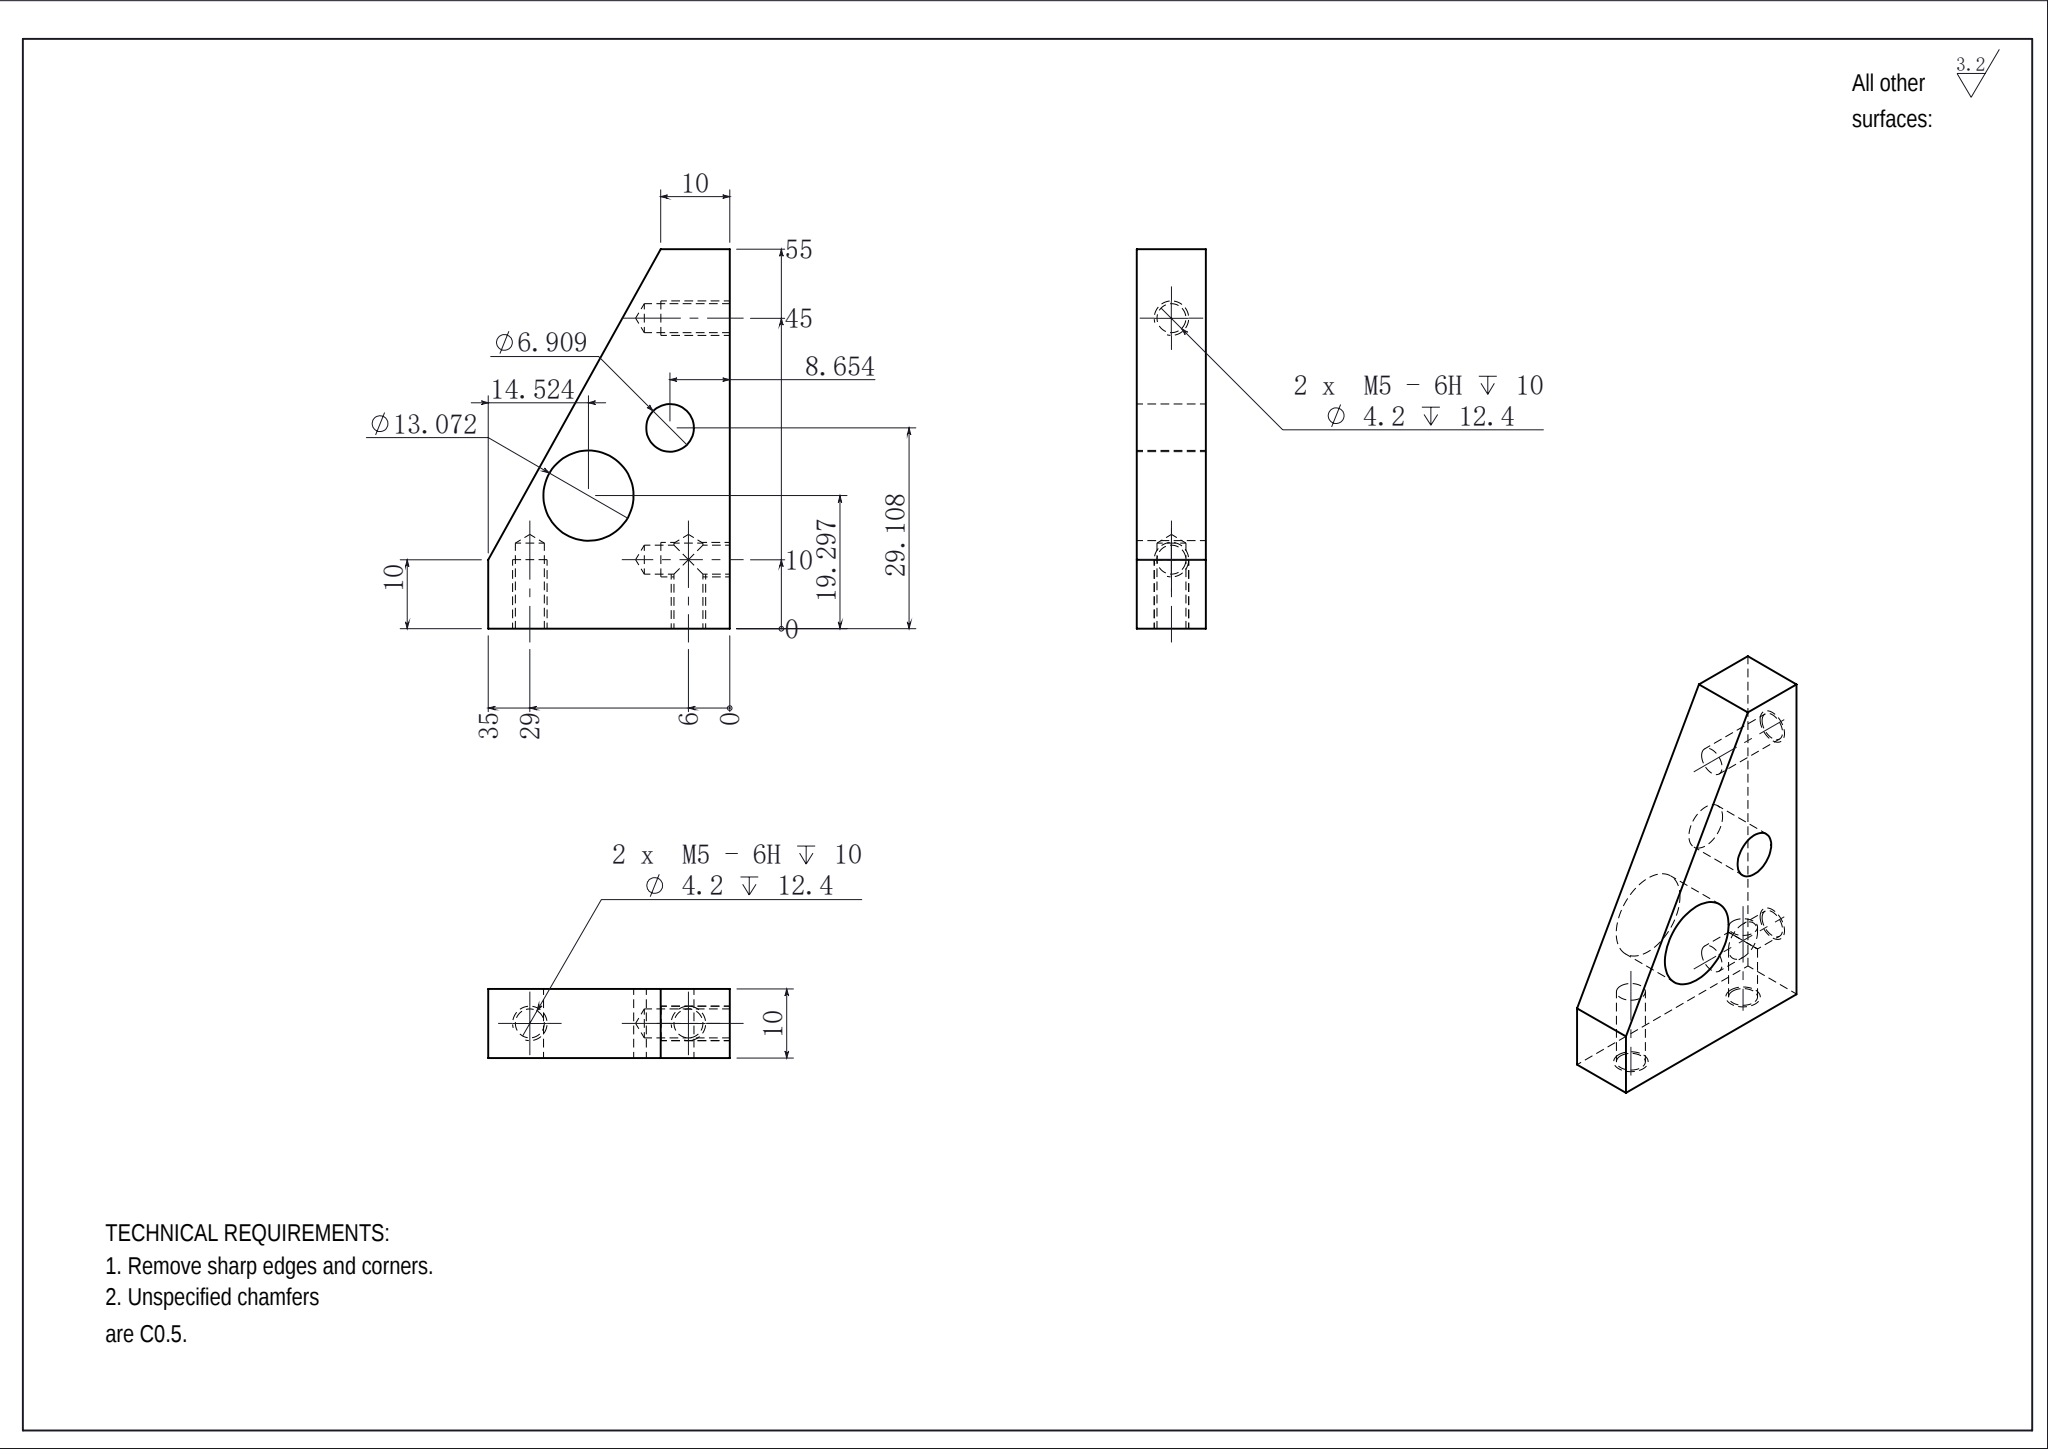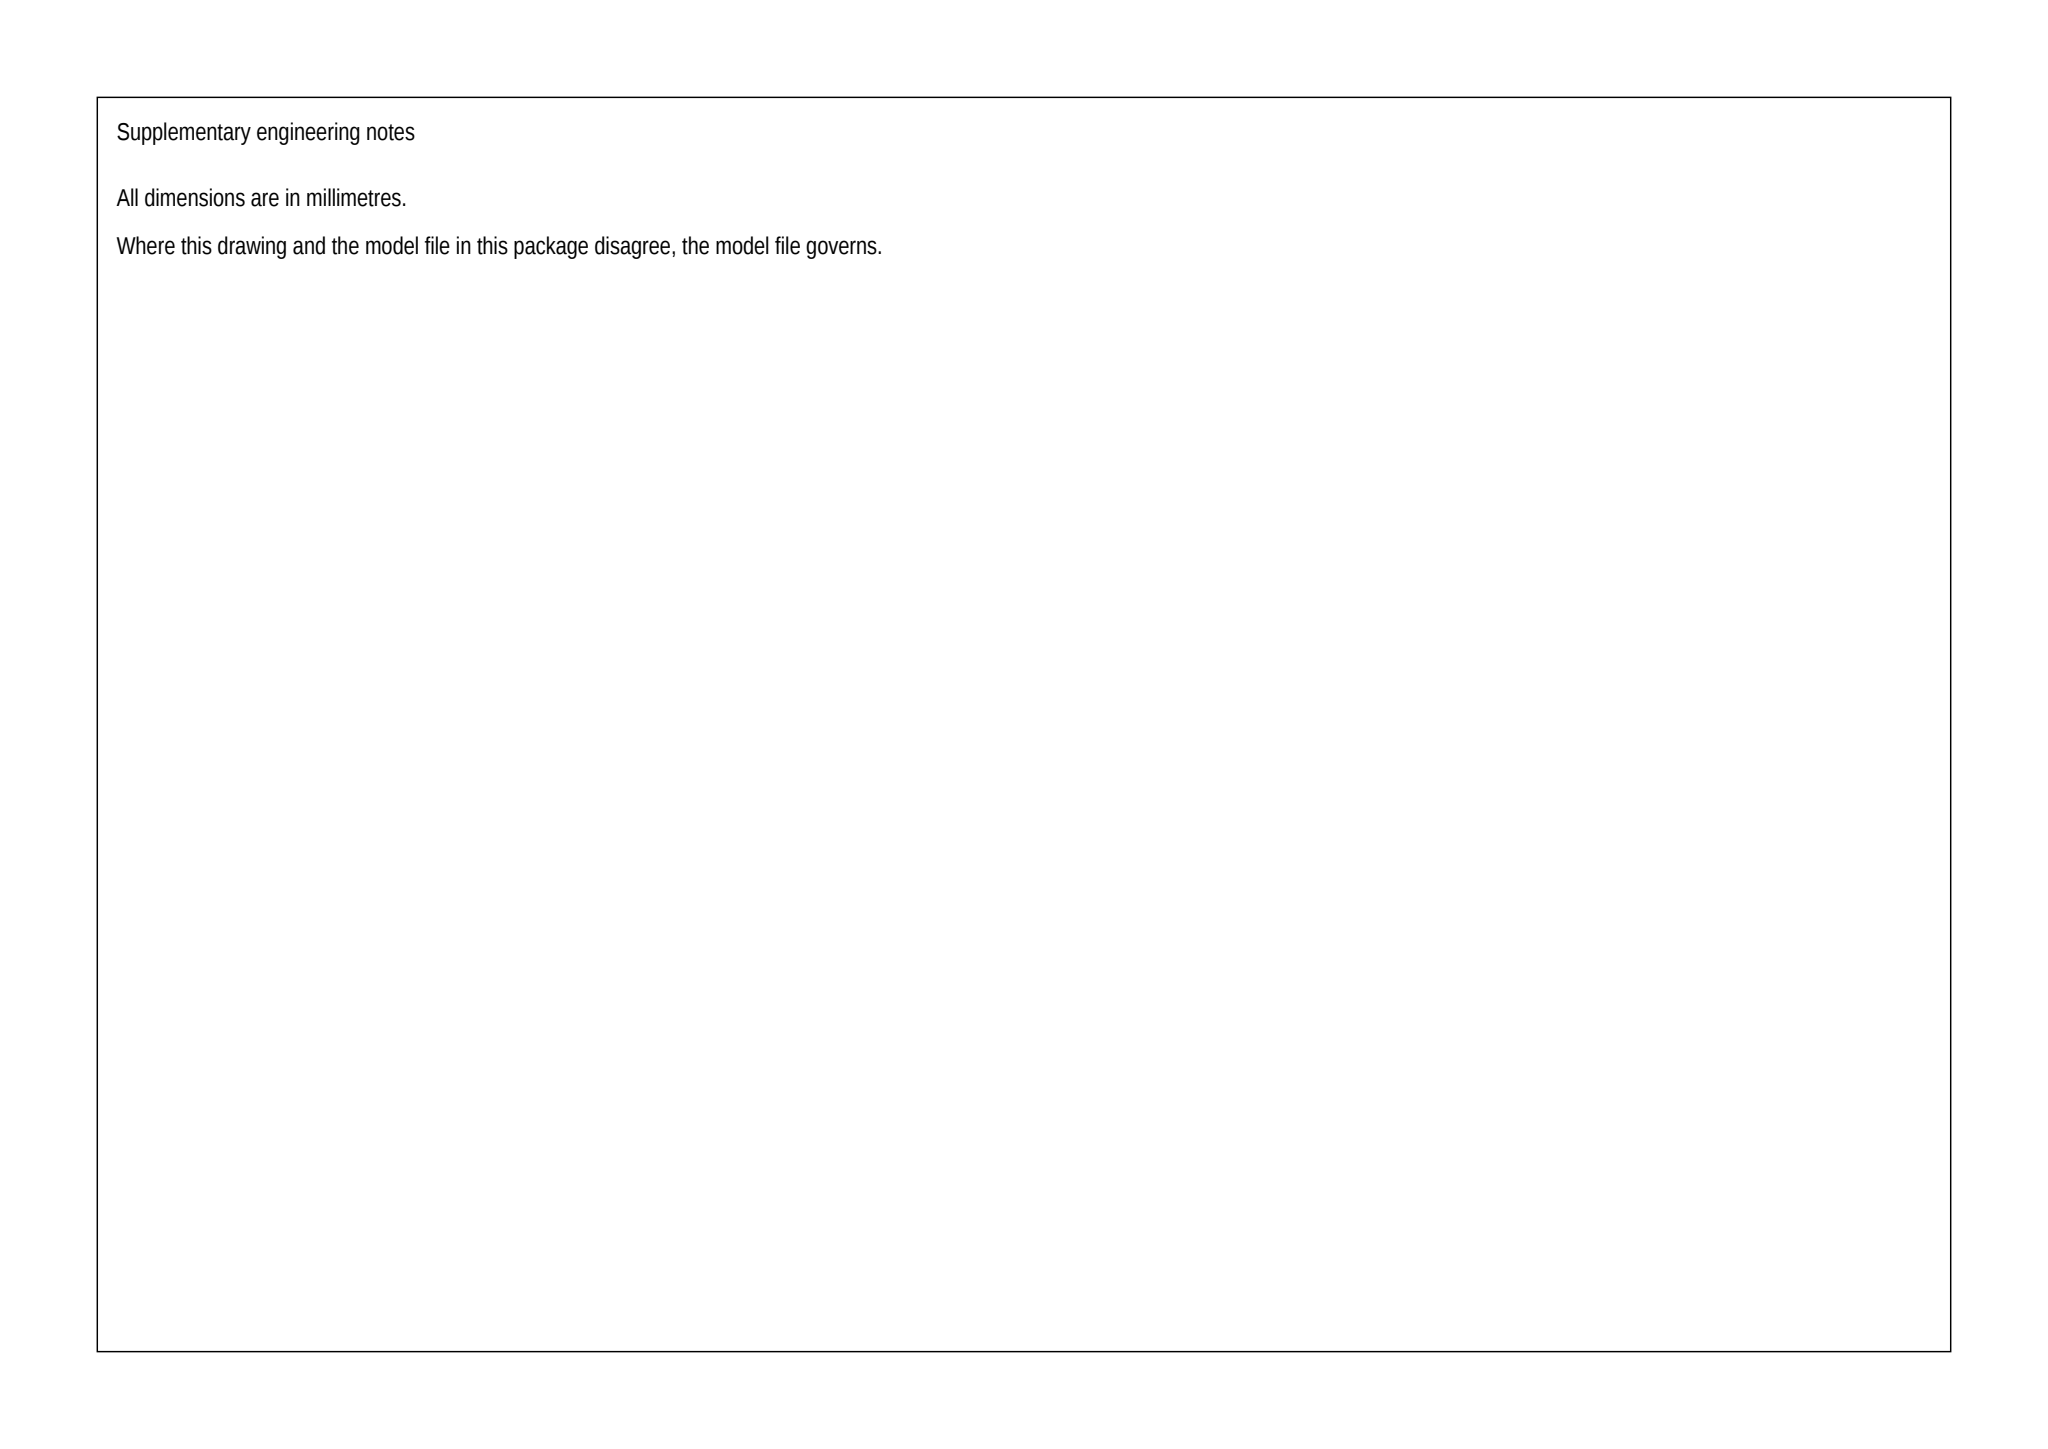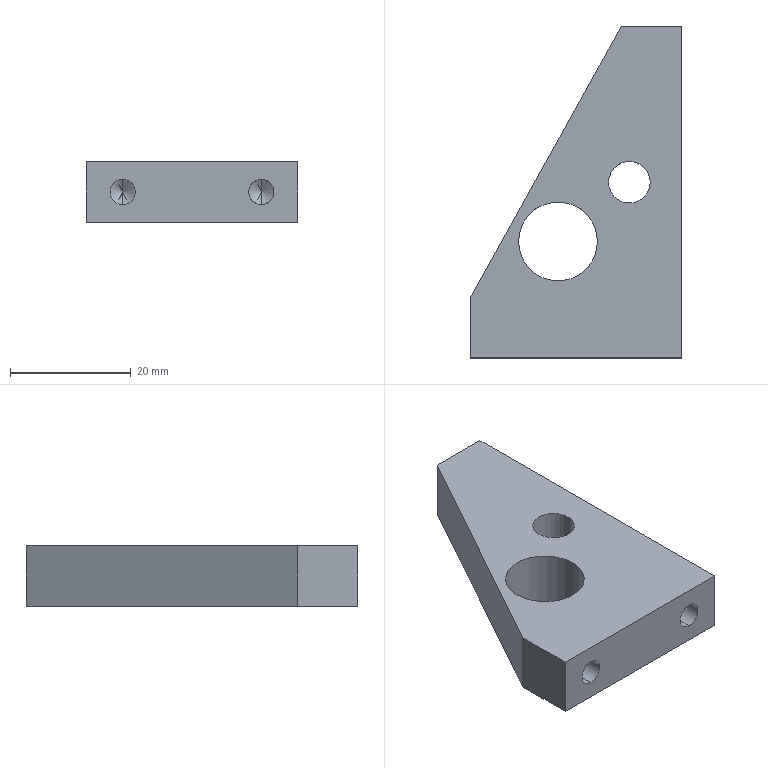Part | SolidWorks | mm | 1 solid | 31 faces | box 35 x 55 x 10 mm | volume 11247 mm3 | cylinder 16 | cone 8 | plane 7 | commonest cylinder face diameters 4.2 x12 13.072 x2 6.909 x2
build123d program:
from build123d import *

# Parameters (mm, degrees)
BOSS_EXTRUDE1_DEPTH   = 5
M5_TAPPED_HOLE1_D     = 4.2
M5_TAPPED_HOLE1_DEPTH = 12.4
M5_TAPPED_HOLE1_TIP   = 1.262
M5_TAPPED_HOLE2_D     = 4.2
M5_TAPPED_HOLE2_DEPTH = 12.4
M5_TAPPED_HOLE2_TIP   = 1.262
SKETCH7_R             = 6.536
SKETCH7_R_2           = 3.454
CUT_EXTRUDE1_DEPTH    = 80


with BuildPart() as part:
    # Sketch1 → Boss-Extrude1 (new, symmetric)
    with BuildSketch(Plane.XY):
        Polygon((0, 0), (0, 55), (-10, 55), (-35, 10), (-35, 0), align=None)
    extrude(amount=BOSS_EXTRUDE1_DEPTH, both=True)

    # M5 Tapped Hole1
    with Locations(Plane(origin=(0, 0, 0), x_dir=(0, 0, -1), z_dir=(1, 0, 0))):
        with Locations((0, 45), (0, 10)):
            Hole(M5_TAPPED_HOLE1_D / 2, depth=M5_TAPPED_HOLE1_DEPTH)
            with Locations((0, 0, -(M5_TAPPED_HOLE1_DEPTH + M5_TAPPED_HOLE1_TIP / 2))):  # 118° drill point
                Cone(0, M5_TAPPED_HOLE1_D / 2, M5_TAPPED_HOLE1_TIP, mode=Mode.SUBTRACT)

    # M5 Tapped Hole2
    with Locations(Plane(origin=(0, 0, 0), x_dir=(-1, 0, 0), z_dir=(0, -1, 0))):
        with Locations((6, 0), (29, 0)):
            Hole(M5_TAPPED_HOLE2_D / 2, depth=M5_TAPPED_HOLE2_DEPTH)
            with Locations((0, 0, -(M5_TAPPED_HOLE2_DEPTH + M5_TAPPED_HOLE2_TIP / 2))):  # 118° drill point
                Cone(0, M5_TAPPED_HOLE2_D / 2, M5_TAPPED_HOLE2_TIP, mode=Mode.SUBTRACT)

    # Sketch7 → Cut-Extrude1 (cut)
    with BuildSketch(Plane.XY.offset(5)):
        with Locations((-20.476, 19.297)):
            Circle(SKETCH7_R)
        with Locations((-8.654, 29.108)):
            Circle(SKETCH7_R_2)
    extrude(amount=-CUT_EXTRUDE1_DEPTH, mode=Mode.SUBTRACT)


solid = part.part
STEP:
#1=CARTESIAN_POINT('',(-27.011,19.297,-5.));
#2=VERTEX_POINT('',#1);
#3=CARTESIAN_POINT('',(-13.94,19.297,-5.));
#4=VERTEX_POINT('',#3);
#5=CARTESIAN_POINT('',(-20.476,19.297,-5.));
#6=DIRECTION('',(0.,0.,1.));
#7=DIRECTION('',(1.,0.,0.));
#8=AXIS2_PLACEMENT_3D('',#5,#6,#7);
#9=CIRCLE('',#8,6.536);
#10=EDGE_CURVE('',#2,#4,#9,.T.);
#11=ORIENTED_EDGE('',*,*,#10,.F.);
#12=CARTESIAN_POINT('',(-27.011,19.297,5.));
#13=VERTEX_POINT('',#12);
#14=CARTESIAN_POINT('',(-27.011,19.297,-75.));
#15=DIRECTION('',(0.,0.,1.));
#16=VECTOR('',#15,1000.);
#17=LINE('',#14,#16);
#18=EDGE_CURVE('',#2,#13,#17,.T.);
#19=ORIENTED_EDGE('',*,*,#18,.T.);
#20=CARTESIAN_POINT('',(-13.94,19.297,5.));
#21=VERTEX_POINT('',#20);
#22=CARTESIAN_POINT('',(-20.476,19.297,5.));
#23=DIRECTION('',(0.,0.,1.));
#24=DIRECTION('',(1.,0.,0.));
#25=AXIS2_PLACEMENT_3D('',#22,#23,#24);
#26=CIRCLE('',#25,6.536);
#27=EDGE_CURVE('',#13,#21,#26,.T.);
#28=ORIENTED_EDGE('',*,*,#27,.T.);
#29=CARTESIAN_POINT('',(-13.94,19.297,-75.));
#30=DIRECTION('',(0.,0.,1.));
#31=VECTOR('',#30,1000.);
#32=LINE('',#29,#31);
#33=EDGE_CURVE('',#4,#21,#32,.T.);
#34=ORIENTED_EDGE('',*,*,#33,.F.);
#35=EDGE_LOOP('',(#11,#19,#28,#34));
#36=FACE_OUTER_BOUND('',#35,.T.);
#37=CARTESIAN_POINT('',(-20.476,19.297,-75.));
#38=DIRECTION('',(0.,0.,1.));
#39=DIRECTION('',(1.,0.,0.));
#40=AXIS2_PLACEMENT_3D('',#37,#38,#39);
#41=CYLINDRICAL_SURFACE('',#40,6.536);
#42=ADVANCED_FACE('',(#36),#41,.F.);
#43=CARTESIAN_POINT('',(-12.108,29.108,-5.));
#44=VERTEX_POINT('',#43);
#45=CARTESIAN_POINT('',(-5.199,29.108,-5.));
#46=VERTEX_POINT('',#45);
#47=CARTESIAN_POINT('',(-8.654,29.108,-5.));
#48=DIRECTION('',(0.,0.,1.));
#49=DIRECTION('',(1.,0.,0.));
#50=AXIS2_PLACEMENT_3D('',#47,#48,#49);
#51=CIRCLE('',#50,3.454);
#52=EDGE_CURVE('',#44,#46,#51,.T.);
#53=ORIENTED_EDGE('',*,*,#52,.F.);
#54=CARTESIAN_POINT('',(-12.108,29.108,5.));
#55=VERTEX_POINT('',#54);
#56=CARTESIAN_POINT('',(-12.108,29.108,-75.));
#57=DIRECTION('',(0.,0.,1.));
#58=VECTOR('',#57,1000.);
#59=LINE('',#56,#58);
#60=EDGE_CURVE('',#44,#55,#59,.T.);
#61=ORIENTED_EDGE('',*,*,#60,.T.);
#62=CARTESIAN_POINT('',(-5.199,29.108,5.));
#63=VERTEX_POINT('',#62);
#64=CARTESIAN_POINT('',(-8.654,29.108,5.));
#65=DIRECTION('',(0.,0.,1.));
#66=DIRECTION('',(1.,0.,0.));
#67=AXIS2_PLACEMENT_3D('',#64,#65,#66);
#68=CIRCLE('',#67,3.454);
#69=EDGE_CURVE('',#55,#63,#68,.T.);
#70=ORIENTED_EDGE('',*,*,#69,.T.);
#71=CARTESIAN_POINT('',(-5.199,29.108,-75.));
#72=DIRECTION('',(0.,0.,1.));
#73=VECTOR('',#72,1000.);
#74=LINE('',#71,#73);
#75=EDGE_CURVE('',#46,#63,#74,.T.);
#76=ORIENTED_EDGE('',*,*,#75,.F.);
#77=EDGE_LOOP('',(#53,#61,#70,#76));
#78=FACE_OUTER_BOUND('',#77,.T.);
#79=CARTESIAN_POINT('',(-8.654,29.108,-75.));
#80=DIRECTION('',(0.,0.,1.));
#81=DIRECTION('',(1.,0.,0.));
#82=AXIS2_PLACEMENT_3D('',#79,#80,#81);
#83=CYLINDRICAL_SURFACE('',#82,3.454);
#84=ADVANCED_FACE('',(#78),#83,.F.);
#85=CARTESIAN_POINT('',(-6.,13.662,0.));
#86=VERTEX_POINT('',#85);
#87=CARTESIAN_POINT('',(-6.,12.4,-2.1));
#88=VERTEX_POINT('',#87);
#89=CARTESIAN_POINT('',(-6.,12.4,-2.1));
#90=DIRECTION('',(0.,-0.515,-0.8572));
#91=VECTOR('',#90,1000.);
#92=LINE('',#89,#91);
#93=EDGE_CURVE('',#86,#88,#92,.T.);
#94=ORIENTED_EDGE('',*,*,#93,.F.);
#95=CARTESIAN_POINT('',(-6.,12.4,2.1));
#96=VERTEX_POINT('',#95);
#97=CARTESIAN_POINT('',(-6.,12.4,2.1));
#98=DIRECTION('',(0.,-0.515,0.8572));
#99=VECTOR('',#98,1000.);
#100=LINE('',#97,#99);
#101=EDGE_CURVE('',#86,#96,#100,.T.);
#102=ORIENTED_EDGE('',*,*,#101,.T.);
#103=CARTESIAN_POINT('',(-6.,12.4,0.));
#104=DIRECTION('',(0.,-1.,0.));
#105=DIRECTION('',(0.,0.,-1.));
#106=AXIS2_PLACEMENT_3D('',#103,#104,#105);
#107=CIRCLE('',#106,2.1);
#108=EDGE_CURVE('',#96,#88,#107,.T.);
#109=ORIENTED_EDGE('',*,*,#108,.T.);
#110=EDGE_LOOP('',(#94,#102,#109));
#111=FACE_OUTER_BOUND('',#110,.T.);
#112=CARTESIAN_POINT('',(-6.,12.4,0.));
#113=DIRECTION('',(0.,-1.,0.));
#114=DIRECTION('',(0.,0.,-1.));
#115=AXIS2_PLACEMENT_3D('',#112,#113,#114);
#116=CONICAL_SURFACE('',#115,2.1,1.03);
#117=ADVANCED_FACE('',(#111),#116,.F.);
#118=ORIENTED_EDGE('',*,*,#108,.F.);
#119=CARTESIAN_POINT('',(-6.,10.,2.1));
#120=VERTEX_POINT('',#119);
#121=CARTESIAN_POINT('',(-6.,0.,2.1));
#122=DIRECTION('',(0.,-1.,0.));
#123=VECTOR('',#122,1000.);
#124=LINE('',#121,#123);
#125=EDGE_CURVE('',#96,#120,#124,.T.);
#126=ORIENTED_EDGE('',*,*,#125,.T.);
#127=CARTESIAN_POINT('',(-6.,10.,-2.1));
#128=VERTEX_POINT('',#127);
#129=CARTESIAN_POINT('',(-6.,10.,-2.1));
#130=CARTESIAN_POINT('',(-10.2,14.2,-2.1));
#131=CARTESIAN_POINT('',(-10.2,14.2,2.1));
#132=CARTESIAN_POINT('',(-6.,10.,2.1));
#133=(BOUNDED_CURVE()B_SPLINE_CURVE(3,(#129,#130,#131,#132),.UNSPECIFIED.,.F.,.F.)B_SPLINE_CURVE_WITH_KNOTS((4,4),(1.571,4.712),.UNSPECIFIED.)CURVE()GEOMETRIC_REPRESENTATION_ITEM()RATIONAL_B_SPLINE_CURVE((1.,0.3333,0.3333,1.))REPRESENTATION_ITEM(''));
#134=EDGE_CURVE('',#128,#120,#133,.T.);
#135=ORIENTED_EDGE('',*,*,#134,.F.);
#136=CARTESIAN_POINT('',(-6.,0.,-2.1));
#137=DIRECTION('',(0.,-1.,0.));
#138=VECTOR('',#137,1000.);
#139=LINE('',#136,#138);
#140=EDGE_CURVE('',#88,#128,#139,.T.);
#141=ORIENTED_EDGE('',*,*,#140,.F.);
#142=EDGE_LOOP('',(#118,#126,#135,#141));
#143=FACE_OUTER_BOUND('',#142,.T.);
#144=CARTESIAN_POINT('',(-6.,0.,0.));
#145=DIRECTION('',(0.,-1.,0.));
#146=DIRECTION('',(0.,0.,-1.));
#147=AXIS2_PLACEMENT_3D('',#144,#145,#146);
#148=CYLINDRICAL_SURFACE('',#147,2.1);
#149=ADVANCED_FACE('',(#143),#148,.F.);
#150=CARTESIAN_POINT('',(-12.4,10.,2.1));
#151=VERTEX_POINT('',#150);
#152=CARTESIAN_POINT('',(-12.4,10.,-2.1));
#153=VERTEX_POINT('',#152);
#154=CARTESIAN_POINT('',(-12.4,10.,-0.));
#155=DIRECTION('',(1.,0.,0.));
#156=DIRECTION('',(0.,0.,-1.));
#157=AXIS2_PLACEMENT_3D('',#154,#155,#156);
#158=CIRCLE('',#157,2.1);
#159=EDGE_CURVE('',#151,#153,#158,.T.);
#160=ORIENTED_EDGE('',*,*,#159,.F.);
#161=CARTESIAN_POINT('',(0.,10.,2.1));
#162=DIRECTION('',(1.,0.,0.));
#163=VECTOR('',#162,1000.);
#164=LINE('',#161,#163);
#165=EDGE_CURVE('',#151,#120,#164,.T.);
#166=ORIENTED_EDGE('',*,*,#165,.T.);
#167=CARTESIAN_POINT('',(-6.,10.,2.1));
#168=CARTESIAN_POINT('',(-10.2,5.8,2.1));
#169=CARTESIAN_POINT('',(-10.2,5.8,-2.1));
#170=CARTESIAN_POINT('',(-6.,10.,-2.1));
#171=(BOUNDED_CURVE()B_SPLINE_CURVE(3,(#167,#168,#169,#170),.UNSPECIFIED.,.F.,.F.)B_SPLINE_CURVE_WITH_KNOTS((4,4),(1.571,4.712),.UNSPECIFIED.)CURVE()GEOMETRIC_REPRESENTATION_ITEM()RATIONAL_B_SPLINE_CURVE((1.,0.3333,0.3333,1.))REPRESENTATION_ITEM(''));
#172=EDGE_CURVE('',#120,#128,#171,.T.);
#173=ORIENTED_EDGE('',*,*,#172,.T.);
#174=CARTESIAN_POINT('',(0.,10.,-2.1));
#175=DIRECTION('',(1.,0.,0.));
#176=VECTOR('',#175,1000.);
#177=LINE('',#174,#176);
#178=EDGE_CURVE('',#153,#128,#177,.T.);
#179=ORIENTED_EDGE('',*,*,#178,.F.);
#180=EDGE_LOOP('',(#160,#166,#173,#179));
#181=FACE_OUTER_BOUND('',#180,.T.);
#182=CARTESIAN_POINT('',(0.,10.,-0.));
#183=DIRECTION('',(1.,0.,0.));
#184=DIRECTION('',(0.,0.,-1.));
#185=AXIS2_PLACEMENT_3D('',#182,#183,#184);
#186=CYLINDRICAL_SURFACE('',#185,2.1);
#187=ADVANCED_FACE('',(#181),#186,.F.);
#188=CARTESIAN_POINT('',(-13.662,10.,-0.));
#189=VERTEX_POINT('',#188);
#190=CARTESIAN_POINT('',(-12.4,10.,-2.1));
#191=DIRECTION('',(0.515,0.,-0.8572));
#192=VECTOR('',#191,1000.);
#193=LINE('',#190,#192);
#194=EDGE_CURVE('',#189,#153,#193,.T.);
#195=ORIENTED_EDGE('',*,*,#194,.F.);
#196=CARTESIAN_POINT('',(-12.4,10.,2.1));
#197=DIRECTION('',(0.515,0.,0.8572));
#198=VECTOR('',#197,1000.);
#199=LINE('',#196,#198);
#200=EDGE_CURVE('',#189,#151,#199,.T.);
#201=ORIENTED_EDGE('',*,*,#200,.T.);
#202=ORIENTED_EDGE('',*,*,#159,.T.);
#203=EDGE_LOOP('',(#195,#201,#202));
#204=FACE_OUTER_BOUND('',#203,.T.);
#205=CARTESIAN_POINT('',(-12.4,10.,-0.));
#206=DIRECTION('',(1.,0.,0.));
#207=DIRECTION('',(0.,0.,-1.));
#208=AXIS2_PLACEMENT_3D('',#205,#206,#207);
#209=CONICAL_SURFACE('',#208,2.1,1.03);
#210=ADVANCED_FACE('',(#204),#209,.F.);
#211=ORIENTED_EDGE('',*,*,#172,.F.);
#212=CARTESIAN_POINT('',(-6.,-0.,2.1));
#213=VERTEX_POINT('',#212);
#214=CARTESIAN_POINT('',(-6.,0.,2.1));
#215=DIRECTION('',(0.,-1.,0.));
#216=VECTOR('',#215,1000.);
#217=LINE('',#214,#216);
#218=EDGE_CURVE('',#120,#213,#217,.T.);
#219=ORIENTED_EDGE('',*,*,#218,.T.);
#220=CARTESIAN_POINT('',(-6.,-0.,-2.1));
#221=VERTEX_POINT('',#220);
#222=CARTESIAN_POINT('',(-6.,-0.,0.));
#223=DIRECTION('',(0.,-1.,0.));
#224=DIRECTION('',(0.,0.,-1.));
#225=AXIS2_PLACEMENT_3D('',#222,#223,#224);
#226=CIRCLE('',#225,2.1);
#227=EDGE_CURVE('',#213,#221,#226,.T.);
#228=ORIENTED_EDGE('',*,*,#227,.T.);
#229=CARTESIAN_POINT('',(-6.,0.,-2.1));
#230=DIRECTION('',(0.,-1.,0.));
#231=VECTOR('',#230,1000.);
#232=LINE('',#229,#231);
#233=EDGE_CURVE('',#128,#221,#232,.T.);
#234=ORIENTED_EDGE('',*,*,#233,.F.);
#235=EDGE_LOOP('',(#211,#219,#228,#234));
#236=FACE_OUTER_BOUND('',#235,.T.);
#237=CARTESIAN_POINT('',(-6.,0.,0.));
#238=DIRECTION('',(0.,-1.,0.));
#239=DIRECTION('',(0.,0.,-1.));
#240=AXIS2_PLACEMENT_3D('',#237,#238,#239);
#241=CYLINDRICAL_SURFACE('',#240,2.1);
#242=ADVANCED_FACE('',(#236),#241,.F.);
#243=CARTESIAN_POINT('',(-29.,12.4,2.1));
#244=VERTEX_POINT('',#243);
#245=CARTESIAN_POINT('',(-29.,12.4,-2.1));
#246=VERTEX_POINT('',#245);
#247=CARTESIAN_POINT('',(-29.,12.4,0.));
#248=DIRECTION('',(0.,-1.,0.));
#249=DIRECTION('',(0.,0.,-1.));
#250=AXIS2_PLACEMENT_3D('',#247,#248,#249);
#251=CIRCLE('',#250,2.1);
#252=EDGE_CURVE('',#244,#246,#251,.T.);
#253=ORIENTED_EDGE('',*,*,#252,.F.);
#254=CARTESIAN_POINT('',(-29.,-0.,2.1));
#255=VERTEX_POINT('',#254);
#256=CARTESIAN_POINT('',(-29.,0.,2.1));
#257=DIRECTION('',(0.,-1.,0.));
#258=VECTOR('',#257,1000.);
#259=LINE('',#256,#258);
#260=EDGE_CURVE('',#244,#255,#259,.T.);
#261=ORIENTED_EDGE('',*,*,#260,.T.);
#262=CARTESIAN_POINT('',(-29.,-0.,-2.1));
#263=VERTEX_POINT('',#262);
#264=CARTESIAN_POINT('',(-29.,-0.,0.));
#265=DIRECTION('',(0.,-1.,0.));
#266=DIRECTION('',(0.,0.,-1.));
#267=AXIS2_PLACEMENT_3D('',#264,#265,#266);
#268=CIRCLE('',#267,2.1);
#269=EDGE_CURVE('',#255,#263,#268,.T.);
#270=ORIENTED_EDGE('',*,*,#269,.T.);
#271=CARTESIAN_POINT('',(-29.,0.,-2.1));
#272=DIRECTION('',(0.,-1.,0.));
#273=VECTOR('',#272,1000.);
#274=LINE('',#271,#273);
#275=EDGE_CURVE('',#246,#263,#274,.T.);
#276=ORIENTED_EDGE('',*,*,#275,.F.);
#277=EDGE_LOOP('',(#253,#261,#270,#276));
#278=FACE_OUTER_BOUND('',#277,.T.);
#279=CARTESIAN_POINT('',(-29.,0.,0.));
#280=DIRECTION('',(0.,-1.,0.));
#281=DIRECTION('',(0.,0.,-1.));
#282=AXIS2_PLACEMENT_3D('',#279,#280,#281);
#283=CYLINDRICAL_SURFACE('',#282,2.1);
#284=ADVANCED_FACE('',(#278),#283,.F.);
#285=CARTESIAN_POINT('',(-29.,13.662,0.));
#286=VERTEX_POINT('',#285);
#287=CARTESIAN_POINT('',(-29.,12.4,-2.1));
#288=DIRECTION('',(0.,-0.515,-0.8572));
#289=VECTOR('',#288,1000.);
#290=LINE('',#287,#289);
#291=EDGE_CURVE('',#286,#246,#290,.T.);
#292=ORIENTED_EDGE('',*,*,#291,.F.);
#293=CARTESIAN_POINT('',(-29.,12.4,2.1));
#294=DIRECTION('',(0.,-0.515,0.8572));
#295=VECTOR('',#294,1000.);
#296=LINE('',#293,#295);
#297=EDGE_CURVE('',#286,#244,#296,.T.);
#298=ORIENTED_EDGE('',*,*,#297,.T.);
#299=ORIENTED_EDGE('',*,*,#252,.T.);
#300=EDGE_LOOP('',(#292,#298,#299));
#301=FACE_OUTER_BOUND('',#300,.T.);
#302=CARTESIAN_POINT('',(-29.,12.4,0.));
#303=DIRECTION('',(0.,-1.,0.));
#304=DIRECTION('',(0.,0.,-1.));
#305=AXIS2_PLACEMENT_3D('',#302,#303,#304);
#306=CONICAL_SURFACE('',#305,2.1,1.03);
#307=ADVANCED_FACE('',(#301),#306,.F.);
#308=CARTESIAN_POINT('',(-12.4,45.,2.1));
#309=VERTEX_POINT('',#308);
#310=CARTESIAN_POINT('',(-12.4,45.,-2.1));
#311=VERTEX_POINT('',#310);
#312=CARTESIAN_POINT('',(-12.4,45.,0.));
#313=DIRECTION('',(1.,0.,0.));
#314=DIRECTION('',(0.,0.,-1.));
#315=AXIS2_PLACEMENT_3D('',#312,#313,#314);
#316=CIRCLE('',#315,2.1);
#317=EDGE_CURVE('',#309,#311,#316,.T.);
#318=ORIENTED_EDGE('',*,*,#317,.F.);
#319=CARTESIAN_POINT('',(-0.,45.,2.1));
#320=VERTEX_POINT('',#319);
#321=CARTESIAN_POINT('',(0.,45.,2.1));
#322=DIRECTION('',(1.,0.,0.));
#323=VECTOR('',#322,1000.);
#324=LINE('',#321,#323);
#325=EDGE_CURVE('',#309,#320,#324,.T.);
#326=ORIENTED_EDGE('',*,*,#325,.T.);
#327=CARTESIAN_POINT('',(-0.,45.,-2.1));
#328=VERTEX_POINT('',#327);
#329=CARTESIAN_POINT('',(-0.,45.,0.));
#330=DIRECTION('',(1.,0.,0.));
#331=DIRECTION('',(0.,0.,-1.));
#332=AXIS2_PLACEMENT_3D('',#329,#330,#331);
#333=CIRCLE('',#332,2.1);
#334=EDGE_CURVE('',#320,#328,#333,.T.);
#335=ORIENTED_EDGE('',*,*,#334,.T.);
#336=CARTESIAN_POINT('',(0.,45.,-2.1));
#337=DIRECTION('',(1.,0.,0.));
#338=VECTOR('',#337,1000.);
#339=LINE('',#336,#338);
#340=EDGE_CURVE('',#311,#328,#339,.T.);
#341=ORIENTED_EDGE('',*,*,#340,.F.);
#342=EDGE_LOOP('',(#318,#326,#335,#341));
#343=FACE_OUTER_BOUND('',#342,.T.);
#344=CARTESIAN_POINT('',(0.,45.,0.));
#345=DIRECTION('',(1.,0.,0.));
#346=DIRECTION('',(0.,0.,-1.));
#347=AXIS2_PLACEMENT_3D('',#344,#345,#346);
#348=CYLINDRICAL_SURFACE('',#347,2.1);
#349=ADVANCED_FACE('',(#343),#348,.F.);
#350=CARTESIAN_POINT('',(-13.662,45.,0.));
#351=VERTEX_POINT('',#350);
#352=CARTESIAN_POINT('',(-12.4,45.,-2.1));
#353=DIRECTION('',(0.515,0.,-0.8572));
#354=VECTOR('',#353,1000.);
#355=LINE('',#352,#354);
#356=EDGE_CURVE('',#351,#311,#355,.T.);
#357=ORIENTED_EDGE('',*,*,#356,.F.);
#358=CARTESIAN_POINT('',(-12.4,45.,2.1));
#359=DIRECTION('',(0.515,0.,0.8572));
#360=VECTOR('',#359,1000.);
#361=LINE('',#358,#360);
#362=EDGE_CURVE('',#351,#309,#361,.T.);
#363=ORIENTED_EDGE('',*,*,#362,.T.);
#364=ORIENTED_EDGE('',*,*,#317,.T.);
#365=EDGE_LOOP('',(#357,#363,#364));
#366=FACE_OUTER_BOUND('',#365,.T.);
#367=CARTESIAN_POINT('',(-12.4,45.,0.));
#368=DIRECTION('',(1.,0.,0.));
#369=DIRECTION('',(0.,0.,-1.));
#370=AXIS2_PLACEMENT_3D('',#367,#368,#369);
#371=CONICAL_SURFACE('',#370,2.1,1.03);
#372=ADVANCED_FACE('',(#366),#371,.F.);
#373=CARTESIAN_POINT('',(-6.,10.,-2.1));
#374=CARTESIAN_POINT('',(-1.8,5.8,-2.1));
#375=CARTESIAN_POINT('',(-1.8,5.8,2.1));
#376=CARTESIAN_POINT('',(-6.,10.,2.1));
#377=(BOUNDED_CURVE()B_SPLINE_CURVE(3,(#373,#374,#375,#376),.UNSPECIFIED.,.F.,.F.)B_SPLINE_CURVE_WITH_KNOTS((4,4),(4.712,7.854),.UNSPECIFIED.)CURVE()GEOMETRIC_REPRESENTATION_ITEM()RATIONAL_B_SPLINE_CURVE((1.,0.3333,0.3333,1.))REPRESENTATION_ITEM(''));
#378=EDGE_CURVE('',#128,#120,#377,.T.);
#379=ORIENTED_EDGE('',*,*,#378,.T.);
#380=CARTESIAN_POINT('',(-0.,10.,2.1));
#381=VERTEX_POINT('',#380);
#382=CARTESIAN_POINT('',(0.,10.,2.1));
#383=DIRECTION('',(1.,0.,0.));
#384=VECTOR('',#383,1000.);
#385=LINE('',#382,#384);
#386=EDGE_CURVE('',#120,#381,#385,.T.);
#387=ORIENTED_EDGE('',*,*,#386,.T.);
#388=CARTESIAN_POINT('',(-0.,10.,-2.1));
#389=VERTEX_POINT('',#388);
#390=CARTESIAN_POINT('',(-0.,10.,-0.));
#391=DIRECTION('',(1.,0.,0.));
#392=DIRECTION('',(0.,0.,-1.));
#393=AXIS2_PLACEMENT_3D('',#390,#391,#392);
#394=CIRCLE('',#393,2.1);
#395=EDGE_CURVE('',#381,#389,#394,.T.);
#396=ORIENTED_EDGE('',*,*,#395,.T.);
#397=CARTESIAN_POINT('',(0.,10.,-2.1));
#398=DIRECTION('',(1.,0.,0.));
#399=VECTOR('',#398,1000.);
#400=LINE('',#397,#399);
#401=EDGE_CURVE('',#128,#389,#400,.T.);
#402=ORIENTED_EDGE('',*,*,#401,.F.);
#403=EDGE_LOOP('',(#379,#387,#396,#402));
#404=FACE_OUTER_BOUND('',#403,.T.);
#405=CARTESIAN_POINT('',(0.,10.,-0.));
#406=DIRECTION('',(1.,0.,0.));
#407=DIRECTION('',(0.,0.,-1.));
#408=AXIS2_PLACEMENT_3D('',#405,#406,#407);
#409=CYLINDRICAL_SURFACE('',#408,2.1);
#410=ADVANCED_FACE('',(#404),#409,.F.);
#411=ORIENTED_EDGE('',*,*,#386,.F.);
#412=CARTESIAN_POINT('',(-6.,10.,2.1));
#413=CARTESIAN_POINT('',(-1.8,14.2,2.1));
#414=CARTESIAN_POINT('',(-1.8,14.2,-2.1));
#415=CARTESIAN_POINT('',(-6.,10.,-2.1));
#416=(BOUNDED_CURVE()B_SPLINE_CURVE(3,(#412,#413,#414,#415),.UNSPECIFIED.,.F.,.F.)B_SPLINE_CURVE_WITH_KNOTS((4,4),(4.712,7.854),.UNSPECIFIED.)CURVE()GEOMETRIC_REPRESENTATION_ITEM()RATIONAL_B_SPLINE_CURVE((1.,0.3333,0.3333,1.))REPRESENTATION_ITEM(''));
#417=EDGE_CURVE('',#120,#128,#416,.T.);
#418=ORIENTED_EDGE('',*,*,#417,.T.);
#419=ORIENTED_EDGE('',*,*,#401,.T.);
#420=CARTESIAN_POINT('',(-0.,10.,-0.));
#421=DIRECTION('',(1.,0.,0.));
#422=DIRECTION('',(0.,0.,-1.));
#423=AXIS2_PLACEMENT_3D('',#420,#421,#422);
#424=CIRCLE('',#423,2.1);
#425=EDGE_CURVE('',#389,#381,#424,.T.);
#426=ORIENTED_EDGE('',*,*,#425,.T.);
#427=EDGE_LOOP('',(#411,#418,#419,#426));
#428=FACE_OUTER_BOUND('',#427,.T.);
#429=CARTESIAN_POINT('',(0.,10.,-0.));
#430=DIRECTION('',(1.,0.,0.));
#431=DIRECTION('',(0.,0.,-1.));
#432=AXIS2_PLACEMENT_3D('',#429,#430,#431);
#433=CYLINDRICAL_SURFACE('',#432,2.1);
#434=ADVANCED_FACE('',(#428),#433,.F.);
#435=CARTESIAN_POINT('',(-6.,-0.,0.));
#436=DIRECTION('',(0.,-1.,0.));
#437=DIRECTION('',(0.,0.,-1.));
#438=AXIS2_PLACEMENT_3D('',#435,#436,#437);
#439=CIRCLE('',#438,2.1);
#440=EDGE_CURVE('',#221,#213,#439,.T.);
#441=ORIENTED_EDGE('',*,*,#440,.F.);
#442=ORIENTED_EDGE('',*,*,#227,.F.);
#443=EDGE_LOOP('',(#441,#442));
#444=FACE_BOUND('',#443,.T.);
#445=CARTESIAN_POINT('',(-29.,-0.,0.));
#446=DIRECTION('',(0.,-1.,0.));
#447=DIRECTION('',(0.,0.,-1.));
#448=AXIS2_PLACEMENT_3D('',#445,#446,#447);
#449=CIRCLE('',#448,2.1);
#450=EDGE_CURVE('',#263,#255,#449,.T.);
#451=ORIENTED_EDGE('',*,*,#450,.F.);
#452=ORIENTED_EDGE('',*,*,#269,.F.);
#453=EDGE_LOOP('',(#451,#452));
#454=FACE_BOUND('',#453,.T.);
#455=CARTESIAN_POINT('',(-35.,0.,-5.));
#456=VERTEX_POINT('',#455);
#457=CARTESIAN_POINT('',(0.,0.,-5.));
#458=VERTEX_POINT('',#457);
#459=CARTESIAN_POINT('',(-35.,0.,-5.));
#460=DIRECTION('',(1.,0.,0.));
#461=VECTOR('',#460,1000.);
#462=LINE('',#459,#461);
#463=EDGE_CURVE('',#456,#458,#462,.T.);
#464=ORIENTED_EDGE('',*,*,#463,.T.);
#465=CARTESIAN_POINT('',(0.,0.,5.));
#466=VERTEX_POINT('',#465);
#467=CARTESIAN_POINT('',(0.,0.,5.));
#468=DIRECTION('',(0.,0.,-1.));
#469=VECTOR('',#468,1000.);
#470=LINE('',#467,#469);
#471=EDGE_CURVE('',#466,#458,#470,.T.);
#472=ORIENTED_EDGE('',*,*,#471,.F.);
#473=CARTESIAN_POINT('',(-35.,0.,5.));
#474=VERTEX_POINT('',#473);
#475=CARTESIAN_POINT('',(-35.,0.,5.));
#476=DIRECTION('',(1.,0.,0.));
#477=VECTOR('',#476,1000.);
#478=LINE('',#475,#477);
#479=EDGE_CURVE('',#474,#466,#478,.T.);
#480=ORIENTED_EDGE('',*,*,#479,.F.);
#481=CARTESIAN_POINT('',(-35.,0.,5.));
#482=DIRECTION('',(0.,0.,-1.));
#483=VECTOR('',#482,1000.);
#484=LINE('',#481,#483);
#485=EDGE_CURVE('',#474,#456,#484,.T.);
#486=ORIENTED_EDGE('',*,*,#485,.T.);
#487=EDGE_LOOP('',(#464,#472,#480,#486));
#488=FACE_OUTER_BOUND('',#487,.T.);
#489=CARTESIAN_POINT('',(-35.,0.,5.));
#490=DIRECTION('',(0.,1.,0.));
#491=DIRECTION('',(0.,0.,1.));
#492=AXIS2_PLACEMENT_3D('',#489,#490,#491);
#493=PLANE('',#492);
#494=ADVANCED_FACE('',(#444,#454,#488),#493,.F.);
#495=CARTESIAN_POINT('',(-0.,45.,0.));
#496=DIRECTION('',(1.,0.,0.));
#497=DIRECTION('',(0.,0.,-1.));
#498=AXIS2_PLACEMENT_3D('',#495,#496,#497);
#499=CIRCLE('',#498,2.1);
#500=EDGE_CURVE('',#328,#320,#499,.T.);
#501=ORIENTED_EDGE('',*,*,#500,.F.);
#502=ORIENTED_EDGE('',*,*,#334,.F.);
#503=EDGE_LOOP('',(#501,#502));
#504=FACE_BOUND('',#503,.T.);
#505=ORIENTED_EDGE('',*,*,#425,.F.);
#506=ORIENTED_EDGE('',*,*,#395,.F.);
#507=EDGE_LOOP('',(#505,#506));
#508=FACE_BOUND('',#507,.T.);
#509=CARTESIAN_POINT('',(0.,55.,-5.));
#510=VERTEX_POINT('',#509);
#511=CARTESIAN_POINT('',(0.,0.,-5.));
#512=DIRECTION('',(0.,1.,0.));
#513=VECTOR('',#512,1000.);
#514=LINE('',#511,#513);
#515=EDGE_CURVE('',#458,#510,#514,.T.);
#516=ORIENTED_EDGE('',*,*,#515,.T.);
#517=CARTESIAN_POINT('',(0.,55.,5.));
#518=VERTEX_POINT('',#517);
#519=CARTESIAN_POINT('',(0.,55.,5.));
#520=DIRECTION('',(0.,0.,-1.));
#521=VECTOR('',#520,1000.);
#522=LINE('',#519,#521);
#523=EDGE_CURVE('',#518,#510,#522,.T.);
#524=ORIENTED_EDGE('',*,*,#523,.F.);
#525=CARTESIAN_POINT('',(0.,0.,5.));
#526=DIRECTION('',(0.,1.,0.));
#527=VECTOR('',#526,1000.);
#528=LINE('',#525,#527);
#529=EDGE_CURVE('',#466,#518,#528,.T.);
#530=ORIENTED_EDGE('',*,*,#529,.F.);
#531=ORIENTED_EDGE('',*,*,#471,.T.);
#532=EDGE_LOOP('',(#516,#524,#530,#531));
#533=FACE_OUTER_BOUND('',#532,.T.);
#534=CARTESIAN_POINT('',(0.,0.,5.));
#535=DIRECTION('',(-1.,0.,0.));
#536=DIRECTION('',(0.,0.,1.));
#537=AXIS2_PLACEMENT_3D('',#534,#535,#536);
#538=PLANE('',#537);
#539=ADVANCED_FACE('',(#504,#508,#533),#538,.F.);
#540=CARTESIAN_POINT('',(-10.,55.,-5.));
#541=VERTEX_POINT('',#540);
#542=CARTESIAN_POINT('',(0.,55.,-5.));
#543=DIRECTION('',(-1.,0.,0.));
#544=VECTOR('',#543,1000.);
#545=LINE('',#542,#544);
#546=EDGE_CURVE('',#510,#541,#545,.T.);
#547=ORIENTED_EDGE('',*,*,#546,.T.);
#548=CARTESIAN_POINT('',(-10.,55.,5.));
#549=VERTEX_POINT('',#548);
#550=CARTESIAN_POINT('',(-10.,55.,5.));
#551=DIRECTION('',(0.,0.,-1.));
#552=VECTOR('',#551,1000.);
#553=LINE('',#550,#552);
#554=EDGE_CURVE('',#549,#541,#553,.T.);
#555=ORIENTED_EDGE('',*,*,#554,.F.);
#556=CARTESIAN_POINT('',(0.,55.,5.));
#557=DIRECTION('',(-1.,0.,0.));
#558=VECTOR('',#557,1000.);
#559=LINE('',#556,#558);
#560=EDGE_CURVE('',#518,#549,#559,.T.);
#561=ORIENTED_EDGE('',*,*,#560,.F.);
#562=ORIENTED_EDGE('',*,*,#523,.T.);
#563=EDGE_LOOP('',(#547,#555,#561,#562));
#564=FACE_OUTER_BOUND('',#563,.T.);
#565=CARTESIAN_POINT('',(0.,55.,5.));
#566=DIRECTION('',(0.,-1.,0.));
#567=DIRECTION('',(0.,0.,-1.));
#568=AXIS2_PLACEMENT_3D('',#565,#566,#567);
#569=PLANE('',#568);
#570=ADVANCED_FACE('',(#564),#569,.F.);
#571=CARTESIAN_POINT('',(-35.,10.,-5.));
#572=VERTEX_POINT('',#571);
#573=CARTESIAN_POINT('',(-10.,55.,-5.));
#574=DIRECTION('',(-0.4856,-0.8742,0.));
#575=VECTOR('',#574,1000.);
#576=LINE('',#573,#575);
#577=EDGE_CURVE('',#541,#572,#576,.T.);
#578=ORIENTED_EDGE('',*,*,#577,.T.);
#579=CARTESIAN_POINT('',(-35.,10.,5.));
#580=VERTEX_POINT('',#579);
#581=CARTESIAN_POINT('',(-35.,10.,5.));
#582=DIRECTION('',(0.,0.,-1.));
#583=VECTOR('',#582,1000.);
#584=LINE('',#581,#583);
#585=EDGE_CURVE('',#580,#572,#584,.T.);
#586=ORIENTED_EDGE('',*,*,#585,.F.);
#587=CARTESIAN_POINT('',(-10.,55.,5.));
#588=DIRECTION('',(-0.4856,-0.8742,0.));
#589=VECTOR('',#588,1000.);
#590=LINE('',#587,#589);
#591=EDGE_CURVE('',#549,#580,#590,.T.);
#592=ORIENTED_EDGE('',*,*,#591,.F.);
#593=ORIENTED_EDGE('',*,*,#554,.T.);
#594=EDGE_LOOP('',(#578,#586,#592,#593));
#595=FACE_OUTER_BOUND('',#594,.T.);
#596=CARTESIAN_POINT('',(-10.,55.,5.));
#597=DIRECTION('',(0.8742,-0.4856,0.));
#598=DIRECTION('',(0.4856,0.8742,0.));
#599=AXIS2_PLACEMENT_3D('',#596,#597,#598);
#600=PLANE('',#599);
#601=ADVANCED_FACE('',(#595),#600,.F.);
#602=CARTESIAN_POINT('',(-35.,10.,-5.));
#603=DIRECTION('',(0.,-1.,0.));
#604=VECTOR('',#603,1000.);
#605=LINE('',#602,#604);
#606=EDGE_CURVE('',#572,#456,#605,.T.);
#607=ORIENTED_EDGE('',*,*,#606,.T.);
#608=ORIENTED_EDGE('',*,*,#485,.F.);
#609=CARTESIAN_POINT('',(-35.,10.,5.));
#610=DIRECTION('',(0.,-1.,0.));
#611=VECTOR('',#610,1000.);
#612=LINE('',#609,#611);
#613=EDGE_CURVE('',#580,#474,#612,.T.);
#614=ORIENTED_EDGE('',*,*,#613,.F.);
#615=ORIENTED_EDGE('',*,*,#585,.T.);
#616=EDGE_LOOP('',(#607,#608,#614,#615));
#617=FACE_OUTER_BOUND('',#616,.T.);
#618=CARTESIAN_POINT('',(-35.,10.,5.));
#619=DIRECTION('',(1.,0.,0.));
#620=DIRECTION('',(0.,0.,-1.));
#621=AXIS2_PLACEMENT_3D('',#618,#619,#620);
#622=PLANE('',#621);
#623=ADVANCED_FACE('',(#617),#622,.F.);
#624=CARTESIAN_POINT('',(-20.476,19.297,5.));
#625=DIRECTION('',(0.,0.,1.));
#626=DIRECTION('',(1.,0.,0.));
#627=AXIS2_PLACEMENT_3D('',#624,#625,#626);
#628=CIRCLE('',#627,6.536);
#629=EDGE_CURVE('',#21,#13,#628,.T.);
#630=ORIENTED_EDGE('',*,*,#629,.F.);
#631=ORIENTED_EDGE('',*,*,#27,.F.);
#632=EDGE_LOOP('',(#630,#631));
#633=FACE_BOUND('',#632,.T.);
#634=CARTESIAN_POINT('',(-8.654,29.108,5.));
#635=DIRECTION('',(0.,0.,1.));
#636=DIRECTION('',(1.,0.,0.));
#637=AXIS2_PLACEMENT_3D('',#634,#635,#636);
#638=CIRCLE('',#637,3.454);
#639=EDGE_CURVE('',#63,#55,#638,.T.);
#640=ORIENTED_EDGE('',*,*,#639,.F.);
#641=ORIENTED_EDGE('',*,*,#69,.F.);
#642=EDGE_LOOP('',(#640,#641));
#643=FACE_BOUND('',#642,.T.);
#644=ORIENTED_EDGE('',*,*,#479,.T.);
#645=ORIENTED_EDGE('',*,*,#529,.T.);
#646=ORIENTED_EDGE('',*,*,#560,.T.);
#647=ORIENTED_EDGE('',*,*,#591,.T.);
#648=ORIENTED_EDGE('',*,*,#613,.T.);
#649=EDGE_LOOP('',(#644,#645,#646,#647,#648));
#650=FACE_OUTER_BOUND('',#649,.T.);
#651=CARTESIAN_POINT('',(0.,0.,5.));
#652=DIRECTION('',(0.,0.,1.));
#653=DIRECTION('',(1.,0.,0.));
#654=AXIS2_PLACEMENT_3D('',#651,#652,#653);
#655=PLANE('',#654);
#656=ADVANCED_FACE('',(#633,#643,#650),#655,.T.);
#657=CARTESIAN_POINT('',(-20.476,19.297,-5.));
#658=DIRECTION('',(0.,0.,1.));
#659=DIRECTION('',(1.,0.,0.));
#660=AXIS2_PLACEMENT_3D('',#657,#658,#659);
#661=CIRCLE('',#660,6.536);
#662=EDGE_CURVE('',#4,#2,#661,.T.);
#663=ORIENTED_EDGE('',*,*,#662,.T.);
#664=ORIENTED_EDGE('',*,*,#10,.T.);
#665=EDGE_LOOP('',(#663,#664));
#666=FACE_BOUND('',#665,.T.);
#667=CARTESIAN_POINT('',(-8.654,29.108,-5.));
#668=DIRECTION('',(0.,0.,1.));
#669=DIRECTION('',(1.,0.,0.));
#670=AXIS2_PLACEMENT_3D('',#667,#668,#669);
#671=CIRCLE('',#670,3.454);
#672=EDGE_CURVE('',#46,#44,#671,.T.);
#673=ORIENTED_EDGE('',*,*,#672,.T.);
#674=ORIENTED_EDGE('',*,*,#52,.T.);
#675=EDGE_LOOP('',(#673,#674));
#676=FACE_BOUND('',#675,.T.);
#677=ORIENTED_EDGE('',*,*,#463,.F.);
#678=ORIENTED_EDGE('',*,*,#606,.F.);
#679=ORIENTED_EDGE('',*,*,#577,.F.);
#680=ORIENTED_EDGE('',*,*,#546,.F.);
#681=ORIENTED_EDGE('',*,*,#515,.F.);
#682=EDGE_LOOP('',(#677,#678,#679,#680,#681));
#683=FACE_OUTER_BOUND('',#682,.T.);
#684=CARTESIAN_POINT('',(0.,0.,-5.));
#685=DIRECTION('',(0.,0.,1.));
#686=DIRECTION('',(1.,0.,0.));
#687=AXIS2_PLACEMENT_3D('',#684,#685,#686);
#688=PLANE('',#687);
#689=ADVANCED_FACE('',(#666,#676,#683),#688,.F.);
#690=ORIENTED_EDGE('',*,*,#362,.F.);
#691=ORIENTED_EDGE('',*,*,#356,.T.);
#692=CARTESIAN_POINT('',(-12.4,45.,0.));
#693=DIRECTION('',(1.,0.,0.));
#694=DIRECTION('',(0.,0.,-1.));
#695=AXIS2_PLACEMENT_3D('',#692,#693,#694);
#696=CIRCLE('',#695,2.1);
#697=EDGE_CURVE('',#311,#309,#696,.T.);
#698=ORIENTED_EDGE('',*,*,#697,.T.);
#699=EDGE_LOOP('',(#690,#691,#698));
#700=FACE_OUTER_BOUND('',#699,.T.);
#701=CARTESIAN_POINT('',(-12.4,45.,0.));
#702=DIRECTION('',(1.,0.,0.));
#703=DIRECTION('',(0.,0.,-1.));
#704=AXIS2_PLACEMENT_3D('',#701,#702,#703);
#705=CONICAL_SURFACE('',#704,2.1,1.03);
#706=ADVANCED_FACE('',(#700),#705,.F.);
#707=ORIENTED_EDGE('',*,*,#325,.F.);
#708=ORIENTED_EDGE('',*,*,#697,.F.);
#709=ORIENTED_EDGE('',*,*,#340,.T.);
#710=ORIENTED_EDGE('',*,*,#500,.T.);
#711=EDGE_LOOP('',(#707,#708,#709,#710));
#712=FACE_OUTER_BOUND('',#711,.T.);
#713=CARTESIAN_POINT('',(0.,45.,0.));
#714=DIRECTION('',(1.,0.,0.));
#715=DIRECTION('',(0.,0.,-1.));
#716=AXIS2_PLACEMENT_3D('',#713,#714,#715);
#717=CYLINDRICAL_SURFACE('',#716,2.1);
#718=ADVANCED_FACE('',(#712),#717,.F.);
#719=ORIENTED_EDGE('',*,*,#297,.F.);
#720=ORIENTED_EDGE('',*,*,#291,.T.);
#721=CARTESIAN_POINT('',(-29.,12.4,0.));
#722=DIRECTION('',(0.,-1.,0.));
#723=DIRECTION('',(0.,0.,-1.));
#724=AXIS2_PLACEMENT_3D('',#721,#722,#723);
#725=CIRCLE('',#724,2.1);
#726=EDGE_CURVE('',#246,#244,#725,.T.);
#727=ORIENTED_EDGE('',*,*,#726,.T.);
#728=EDGE_LOOP('',(#719,#720,#727));
#729=FACE_OUTER_BOUND('',#728,.T.);
#730=CARTESIAN_POINT('',(-29.,12.4,0.));
#731=DIRECTION('',(0.,-1.,0.));
#732=DIRECTION('',(0.,0.,-1.));
#733=AXIS2_PLACEMENT_3D('',#730,#731,#732);
#734=CONICAL_SURFACE('',#733,2.1,1.03);
#735=ADVANCED_FACE('',(#729),#734,.F.);
#736=ORIENTED_EDGE('',*,*,#260,.F.);
#737=ORIENTED_EDGE('',*,*,#726,.F.);
#738=ORIENTED_EDGE('',*,*,#275,.T.);
#739=ORIENTED_EDGE('',*,*,#450,.T.);
#740=EDGE_LOOP('',(#736,#737,#738,#739));
#741=FACE_OUTER_BOUND('',#740,.T.);
#742=CARTESIAN_POINT('',(-29.,0.,0.));
#743=DIRECTION('',(0.,-1.,0.));
#744=DIRECTION('',(0.,0.,-1.));
#745=AXIS2_PLACEMENT_3D('',#742,#743,#744);
#746=CYLINDRICAL_SURFACE('',#745,2.1);
#747=ADVANCED_FACE('',(#741),#746,.F.);
#748=ORIENTED_EDGE('',*,*,#218,.F.);
#749=ORIENTED_EDGE('',*,*,#378,.F.);
#750=ORIENTED_EDGE('',*,*,#233,.T.);
#751=ORIENTED_EDGE('',*,*,#440,.T.);
#752=EDGE_LOOP('',(#748,#749,#750,#751));
#753=FACE_OUTER_BOUND('',#752,.T.);
#754=CARTESIAN_POINT('',(-6.,0.,0.));
#755=DIRECTION('',(0.,-1.,0.));
#756=DIRECTION('',(0.,0.,-1.));
#757=AXIS2_PLACEMENT_3D('',#754,#755,#756);
#758=CYLINDRICAL_SURFACE('',#757,2.1);
#759=ADVANCED_FACE('',(#753),#758,.F.);
#760=ORIENTED_EDGE('',*,*,#200,.F.);
#761=ORIENTED_EDGE('',*,*,#194,.T.);
#762=CARTESIAN_POINT('',(-12.4,10.,-0.));
#763=DIRECTION('',(1.,0.,0.));
#764=DIRECTION('',(0.,0.,-1.));
#765=AXIS2_PLACEMENT_3D('',#762,#763,#764);
#766=CIRCLE('',#765,2.1);
#767=EDGE_CURVE('',#153,#151,#766,.T.);
#768=ORIENTED_EDGE('',*,*,#767,.T.);
#769=EDGE_LOOP('',(#760,#761,#768));
#770=FACE_OUTER_BOUND('',#769,.T.);
#771=CARTESIAN_POINT('',(-12.4,10.,-0.));
#772=DIRECTION('',(1.,0.,0.));
#773=DIRECTION('',(0.,0.,-1.));
#774=AXIS2_PLACEMENT_3D('',#771,#772,#773);
#775=CONICAL_SURFACE('',#774,2.1,1.03);
#776=ADVANCED_FACE('',(#770),#775,.F.);
#777=ORIENTED_EDGE('',*,*,#165,.F.);
#778=ORIENTED_EDGE('',*,*,#767,.F.);
#779=ORIENTED_EDGE('',*,*,#178,.T.);
#780=ORIENTED_EDGE('',*,*,#134,.T.);
#781=EDGE_LOOP('',(#777,#778,#779,#780));
#782=FACE_OUTER_BOUND('',#781,.T.);
#783=CARTESIAN_POINT('',(0.,10.,-0.));
#784=DIRECTION('',(1.,0.,0.));
#785=DIRECTION('',(0.,0.,-1.));
#786=AXIS2_PLACEMENT_3D('',#783,#784,#785);
#787=CYLINDRICAL_SURFACE('',#786,2.1);
#788=ADVANCED_FACE('',(#782),#787,.F.);
#789=ORIENTED_EDGE('',*,*,#125,.F.);
#790=CARTESIAN_POINT('',(-6.,12.4,0.));
#791=DIRECTION('',(0.,-1.,0.));
#792=DIRECTION('',(0.,0.,-1.));
#793=AXIS2_PLACEMENT_3D('',#790,#791,#792);
#794=CIRCLE('',#793,2.1);
#795=EDGE_CURVE('',#88,#96,#794,.T.);
#796=ORIENTED_EDGE('',*,*,#795,.F.);
#797=ORIENTED_EDGE('',*,*,#140,.T.);
#798=ORIENTED_EDGE('',*,*,#417,.F.);
#799=EDGE_LOOP('',(#789,#796,#797,#798));
#800=FACE_OUTER_BOUND('',#799,.T.);
#801=CARTESIAN_POINT('',(-6.,0.,0.));
#802=DIRECTION('',(0.,-1.,0.));
#803=DIRECTION('',(0.,0.,-1.));
#804=AXIS2_PLACEMENT_3D('',#801,#802,#803);
#805=CYLINDRICAL_SURFACE('',#804,2.1);
#806=ADVANCED_FACE('',(#800),#805,.F.);
#807=ORIENTED_EDGE('',*,*,#101,.F.);
#808=ORIENTED_EDGE('',*,*,#93,.T.);
#809=ORIENTED_EDGE('',*,*,#795,.T.);
#810=EDGE_LOOP('',(#807,#808,#809));
#811=FACE_OUTER_BOUND('',#810,.T.);
#812=CARTESIAN_POINT('',(-6.,12.4,0.));
#813=DIRECTION('',(0.,-1.,0.));
#814=DIRECTION('',(0.,0.,-1.));
#815=AXIS2_PLACEMENT_3D('',#812,#813,#814);
#816=CONICAL_SURFACE('',#815,2.1,1.03);
#817=ADVANCED_FACE('',(#811),#816,.F.);
#818=ORIENTED_EDGE('',*,*,#60,.F.);
#819=ORIENTED_EDGE('',*,*,#672,.F.);
#820=ORIENTED_EDGE('',*,*,#75,.T.);
#821=ORIENTED_EDGE('',*,*,#639,.T.);
#822=EDGE_LOOP('',(#818,#819,#820,#821));
#823=FACE_OUTER_BOUND('',#822,.T.);
#824=CARTESIAN_POINT('',(-8.654,29.108,-75.));
#825=DIRECTION('',(0.,0.,1.));
#826=DIRECTION('',(1.,0.,0.));
#827=AXIS2_PLACEMENT_3D('',#824,#825,#826);
#828=CYLINDRICAL_SURFACE('',#827,3.454);
#829=ADVANCED_FACE('',(#823),#828,.F.);
#830=ORIENTED_EDGE('',*,*,#18,.F.);
#831=ORIENTED_EDGE('',*,*,#662,.F.);
#832=ORIENTED_EDGE('',*,*,#33,.T.);
#833=ORIENTED_EDGE('',*,*,#629,.T.);
#834=EDGE_LOOP('',(#830,#831,#832,#833));
#835=FACE_OUTER_BOUND('',#834,.T.);
#836=CARTESIAN_POINT('',(-20.476,19.297,-75.));
#837=DIRECTION('',(0.,0.,1.));
#838=DIRECTION('',(1.,0.,0.));
#839=AXIS2_PLACEMENT_3D('',#836,#837,#838);
#840=CYLINDRICAL_SURFACE('',#839,6.536);
#841=ADVANCED_FACE('',(#835),#840,.F.);
#842=CLOSED_SHELL('',(#42,#84,#117,#149,#187,#210,#242,#284,#307,#349,#372,#410,#434,#494,#539,#570,#601,#623,#656,#689,#706,#718,#735,#747,#759,#776,#788,#806,#817,#829,#841));
#843=MANIFOLD_SOLID_BREP('',#842);
#844=CARTESIAN_POINT('',(0.,0.,0.));
#845=DIRECTION('',(0.,0.,1.));
#846=DIRECTION('',(1.,0.,0.));
#847=AXIS2_PLACEMENT_3D('',#844,#845,#846);
#848=(LENGTH_UNIT()NAMED_UNIT(*)SI_UNIT(.MILLI.,.METRE.));
#849=UNCERTAINTY_MEASURE_WITH_UNIT(LENGTH_MEASURE(0.00001),#848,'','');
#850=(NAMED_UNIT(*)PLANE_ANGLE_UNIT()SI_UNIT($,.RADIAN.));
#851=(NAMED_UNIT(*)SI_UNIT($,.STERADIAN.)SOLID_ANGLE_UNIT());
#852=(GEOMETRIC_REPRESENTATION_CONTEXT(3)GLOBAL_UNCERTAINTY_ASSIGNED_CONTEXT((#849))GLOBAL_UNIT_ASSIGNED_CONTEXT((#848,#850,#851))REPRESENTATION_CONTEXT('',''));
#853=ADVANCED_BREP_SHAPE_REPRESENTATION('',(#843,#847),#852);